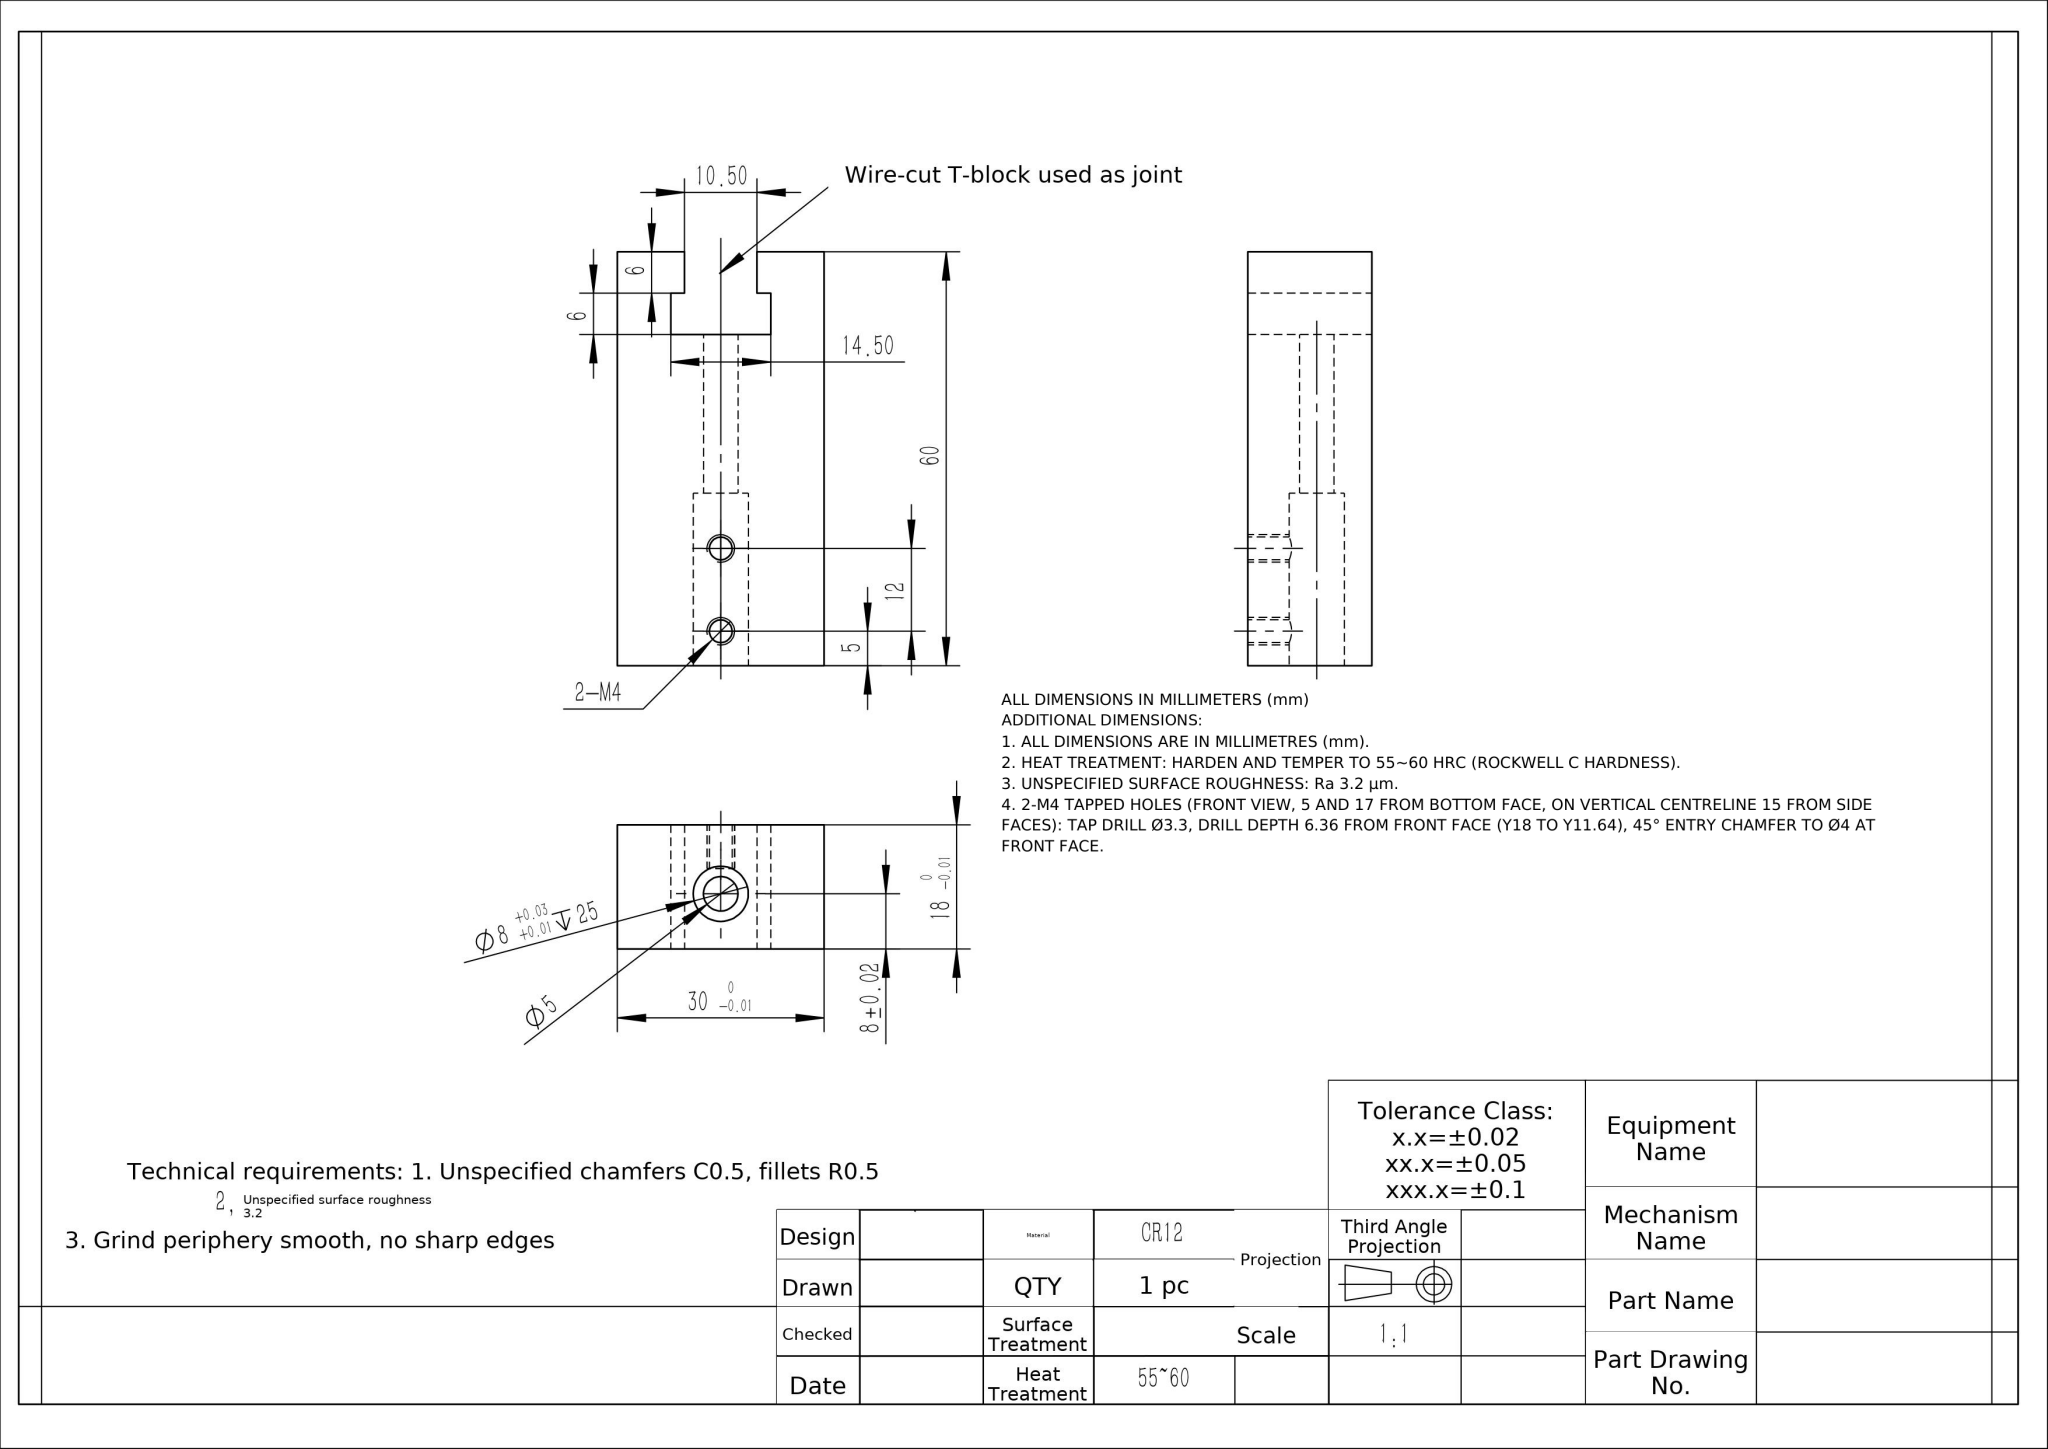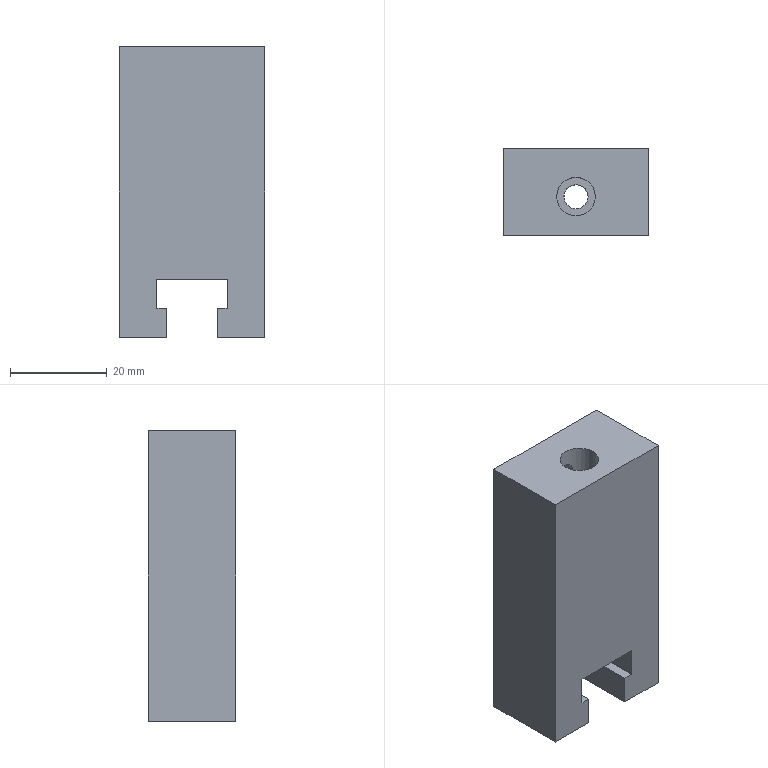Part | NX | mm | Notched Tall Bore Block | 1 solid | 21 faces | box 30 x 18 x 60 mm | volume 27886 mm3 | plane 15 | cylinder 4 | cone 2 | commonest cylinder face diameters 3.3 x2 8 x1 5 x1